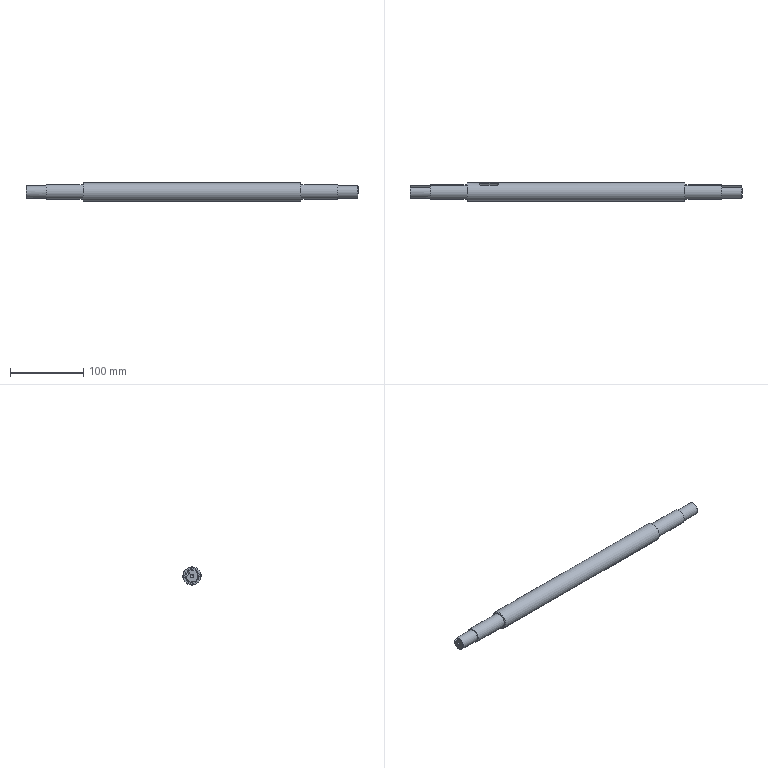Component | SolidWorks | CCD07DriveAxis-1 | 1 solid | 46 faces | box 454 x 25 x 25 mm | volume 187277 mm3 | cylinder 18 | plane 17 | cone 11 | commonest cylinder face diameters 6 x6 5 x4 20 x4 25 x2 17 x2
build123d program:
from build123d import *

# Parameters (mm, degrees)
CUT_EXTRUDE1_DEPTH    = 3.2
CUT_EXTRUDE2_DEPTH    = 3.2
CHAMFER1_SIZE         = 0.5
M6_TAPPED_HOLE1_D     = 5
M6_TAPPED_HOLE1_DEPTH = 20
M6_TAPPED_HOLE1_TIP   = 1.502
M6_TAPPED_HOLE2_D     = 5
M6_TAPPED_HOLE2_DEPTH = 24
M6_TAPPED_HOLE2_TIP   = 1.502


with BuildPart() as part:
    # Sketch1 → Revolve1 (revolve)
    with BuildSketch(Plane.XY, mode=Mode.PRIVATE) as revolve1_sk:
        Polygon((-165.015, 0), (-165.015, 8.5), (-137.015, 8.5), (-137.015, 10), (-87.015, 10), (-87.015, 12.5), (210.985, 12.5), (210.985, 10), (260.985, 10), (260.985, 8.5), (288.985, 8.5), (288.985, 0), align=None)
    revolve(revolve1_sk.sketch.rotate(Axis((-274.431, 0, 0), (1, 0, 0)), 90), axis=Axis((-274.431, 0, 0), (1, 0, 0)))

    # Sketch2 → Cut-Extrude1 (cut)
    with BuildSketch(Plane.XY.offset(8.5)):
        with BuildLine():
            Line((-165.015, 3), (-120.015, 3))
            ThreePointArc((-120.015, 3), (-117.015, 0), (-120.015, -3))
            Line((-120.015, -3), (-165.015, -3))
            ThreePointArc((-165.015, -3), (-168.015, 0), (-165.015, 3))
        make_face()
        with BuildLine():
            Line((288.985, -3), (243.985, -3))
            ThreePointArc((243.985, -3), (240.985, 0), (243.985, 3))
            Line((243.985, 3), (288.985, 3))
            ThreePointArc((288.985, 3), (291.985, 0), (288.985, -3))
        make_face()
    extrude(amount=-CUT_EXTRUDE1_DEPTH, mode=Mode.SUBTRACT)

    # Sketch3 → Cut-Extrude2 (cut)
    with BuildSketch(Plane.XY.offset(12.5)):
        with BuildLine():
            Line((-67.015, 3), (-47.015, 3))
            ThreePointArc((-47.015, 3), (-44.015, 0), (-47.015, -3))
            Line((-47.015, -3), (-67.015, -3))
            ThreePointArc((-67.015, -3), (-70.015, 0), (-67.015, 3))
        make_face()
    extrude(amount=-CUT_EXTRUDE2_DEPTH, mode=Mode.SUBTRACT)

    # Chamfer1
    chamfer1_edges = [part.edges().sort_by_distance(p)[0] for p in [
        (210.985, 0, -12.5),
        (-87.015, 0, -12.5),
        (288.985, 0, -8.5),
        (-165.015, 0, -8.5),
    ]]
    chamfer(chamfer1_edges, length=CHAMFER1_SIZE)

    # M6 Tapped Hole1
    with Locations(Plane.ZY.offset(165.015)):
        with Locations((0, 0)):
            Hole(M6_TAPPED_HOLE1_D / 2, depth=M6_TAPPED_HOLE1_DEPTH)
            with Locations((0, 0, -(M6_TAPPED_HOLE1_DEPTH + M6_TAPPED_HOLE1_TIP / 2))):  # 118° drill point
                Cone(0, M6_TAPPED_HOLE1_D / 2, M6_TAPPED_HOLE1_TIP, mode=Mode.SUBTRACT)

    # M6 Tapped Hole2
    with Locations(Plane(origin=(288.985, 0, 0), x_dir=(0, 0, -1), z_dir=(1, 0, 0))):
        with Locations((0, 0)):
            Hole(M6_TAPPED_HOLE2_D / 2, depth=M6_TAPPED_HOLE2_DEPTH)
            with Locations((0, 0, -(M6_TAPPED_HOLE2_DEPTH + M6_TAPPED_HOLE2_TIP / 2))):  # 118° drill point
                Cone(0, M6_TAPPED_HOLE2_D / 2, M6_TAPPED_HOLE2_TIP, mode=Mode.SUBTRACT)


solid = part.part

# Placed as in the assembly
solid = solid.moved(Location((-179.106, 107.251, -99), (-56.918, 0, 0)))